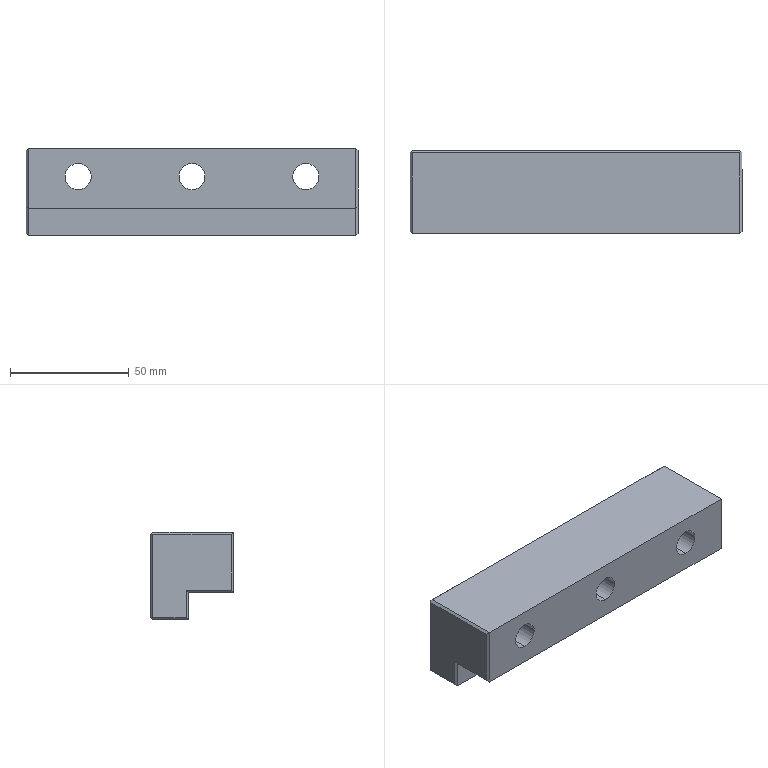Component | SolidWorks | UpperDieShankSeat-1 | 1 solid | 37 faces | box 140 x 35 x 37 mm | volume 135382 mm3 | plane 25 | cylinder 12 | commonest cylinder face diameters 18 x6 11 x6
build123d program:
from build123d import *

# Parameters (mm, degrees)
SKETCH1_W                                        = 140
SKETCH1_H                                        = 140
BOSS_EXTRUDE1_DEPTH                              = 35
SKETCH2_W                                        = 114.165
SKETCH2_H                                        = 44.114
CUT_EXTRUDE1_DEPTH                               = 161.39
SKETCH3_W                                        = 18.069
SKETCH3_H                                        = 21.674
SKETCH3_W_2                                      = 16.574
SKETCH3_H_2                                      = 23.169
CUT_EXTRUDE2_DEPTH                               = 161.39
M10_HEX_SOCKET_HEAD_CAP_SCREW_CBORE1_D           = 11
M10_HEX_SOCKET_HEAD_CAP_SCREW_CBORE1_CBORE_D     = 18
M10_HEX_SOCKET_HEAD_CAP_SCREW_CBORE1_CBORE_DEPTH = 10.6
CHAMFER1_SIZE                                    = 1
CHAMFER2_SIZE                                    = 1
CHAMFER3_SIZE                                    = 1


with BuildPart() as part:
    # Sketch1 → Boss-Extrude1 (new body)
    with BuildSketch(Plane.XY):
        Rectangle(SKETCH1_W, SKETCH1_H)
    extrude(amount=BOSS_EXTRUDE1_DEPTH)

    # Sketch2 → Cut-Extrude1 (cut, through all)
    with BuildSketch(Plane.XZ.offset(70)):
        with Locations((24.082, 18.552)):
            Rectangle(SKETCH2_W, SKETCH2_H)
    extrude(amount=-CUT_EXTRUDE1_DEPTH, mode=Mode.SUBTRACT)

    # Sketch3 → Cut-Extrude2 (cut, through all)
    with BuildSketch(Plane.XZ.offset(70)):
        with Locations((-35.466, 8.163)):
            Rectangle(SKETCH3_W, SKETCH3_H)
        with Locations((35.963, 8.098)):
            Rectangle(SKETCH3_W_2, SKETCH3_H_2)
    extrude(amount=-CUT_EXTRUDE2_DEPTH, mode=Mode.SUBTRACT)

    # M10 Hex Socket Head Cap Screw CBORE1 (through all)
    with Locations(Plane.XY.offset(35)):
        with Locations((-58, 48), (-58, 0), (-58, -48)):
            CounterBoreHole(M10_HEX_SOCKET_HEAD_CAP_SCREW_CBORE1_D / 2, M10_HEX_SOCKET_HEAD_CAP_SCREW_CBORE1_CBORE_D / 2, M10_HEX_SOCKET_HEAD_CAP_SCREW_CBORE1_CBORE_DEPTH)

    # Chamfer1
    chamfer1_edges = [part.edges().sort_by_distance(p)[0] for p in [
        (-33, -70, 27),
        (-38.75, -70, 19),
        (-44.5, -70, 9.5),
        (-57.25, -70, 0),
        (-51.5, -70, 35),
        (-70, -70, 17.5),
    ]]
    chamfer(chamfer1_edges, length=CHAMFER1_SIZE)

    # Chamfer2
    chamfer2_edges = [part.edges().sort_by_distance(p)[0] for p in [
        (-51.5, 70, 35),
        (-33, 70, 27),
        (-57.25, 70, 0),
        (-44.5, 70, 9.5),
        (-38.75, 70, 19),
        (-70, 70, 17.5),
    ]]
    chamfer(chamfer2_edges, length=CHAMFER2_SIZE)

    # Chamfer3
    chamfer3_edges = [part.edges().sort_by_distance(p)[0] for p in [
        (-33, 0, 35),
        (-70, 0, 35),
    ]]
    chamfer(chamfer3_edges, length=CHAMFER3_SIZE)


solid = part.part

# Placed as in the assembly
solid = solid.moved(Location((-177.951, 643.269, 5), (-90, 0, 90)))
STEP:
#1=COLOUR_RGB('',0.7922,0.8196,0.9333);
#2=FILL_AREA_STYLE_COLOUR('',#1);
#3=FILL_AREA_STYLE('',(#2));
#4=SURFACE_STYLE_FILL_AREA(#3);
#5=SURFACE_SIDE_STYLE('',(#4));
#6=SURFACE_STYLE_USAGE(.BOTH.,#5);
#7=PRESENTATION_STYLE_ASSIGNMENT((#6));
#8=CARTESIAN_POINT('',(-8.896,26.286,2.835));
#9=VERTEX_POINT('',#8);
#10=CARTESIAN_POINT('',(-8.896,26.286,2.126));
#11=VERTEX_POINT('',#10);
#12=CARTESIAN_POINT('',(-8.896,26.286,2.48));
#13=DIRECTION('',(-0.,1.,0.));
#14=DIRECTION('',(0.,0.,-1.));
#15=AXIS2_PLACEMENT_3D('',#12,#13,#14);
#16=CIRCLE('',#15,0.3543);
#17=EDGE_CURVE('',#9,#11,#16,.T.);
#18=ORIENTED_EDGE('',*,*,#17,.F.);
#19=CARTESIAN_POINT('',(-8.896,26.704,2.835));
#20=VERTEX_POINT('',#19);
#21=CARTESIAN_POINT('',(-8.896,26.704,2.835));
#22=DIRECTION('',(-0.,1.,0.));
#23=VECTOR('',#22,39.37);
#24=LINE('',#21,#23);
#25=EDGE_CURVE('',#9,#20,#24,.T.);
#26=ORIENTED_EDGE('',*,*,#25,.T.);
#27=CARTESIAN_POINT('',(-8.896,26.704,2.126));
#28=VERTEX_POINT('',#27);
#29=CARTESIAN_POINT('',(-8.896,26.704,2.48));
#30=DIRECTION('',(-0.,1.,0.));
#31=DIRECTION('',(0.,0.,-1.));
#32=AXIS2_PLACEMENT_3D('',#29,#30,#31);
#33=CIRCLE('',#32,0.3543);
#34=EDGE_CURVE('',#20,#28,#33,.T.);
#35=ORIENTED_EDGE('',*,*,#34,.T.);
#36=CARTESIAN_POINT('',(-8.896,26.704,2.126));
#37=DIRECTION('',(-0.,1.,0.));
#38=VECTOR('',#37,39.37);
#39=LINE('',#36,#38);
#40=EDGE_CURVE('',#11,#28,#39,.T.);
#41=ORIENTED_EDGE('',*,*,#40,.F.);
#42=EDGE_LOOP('',(#18,#26,#35,#41));
#43=FACE_OUTER_BOUND('',#42,.T.);
#44=CARTESIAN_POINT('',(-8.896,26.704,2.48));
#45=DIRECTION('',(-0.,1.,0.));
#46=DIRECTION('',(0.,0.,-1.));
#47=AXIS2_PLACEMENT_3D('',#44,#45,#46);
#48=CYLINDRICAL_SURFACE('',#47,0.3543);
#49=ADVANCED_FACE('',(#43),#48,.F.);
#50=CARTESIAN_POINT('',(-8.896,25.326,2.697));
#51=VERTEX_POINT('',#50);
#52=CARTESIAN_POINT('',(-8.896,25.326,2.264));
#53=VERTEX_POINT('',#52);
#54=CARTESIAN_POINT('',(-8.896,25.326,2.48));
#55=DIRECTION('',(-0.,1.,0.));
#56=DIRECTION('',(0.,0.,-1.));
#57=AXIS2_PLACEMENT_3D('',#54,#55,#56);
#58=CIRCLE('',#57,0.2165);
#59=EDGE_CURVE('',#51,#53,#58,.T.);
#60=ORIENTED_EDGE('',*,*,#59,.F.);
#61=CARTESIAN_POINT('',(-8.896,26.286,2.697));
#62=VERTEX_POINT('',#61);
#63=CARTESIAN_POINT('',(-8.896,26.704,2.697));
#64=DIRECTION('',(-0.,1.,0.));
#65=VECTOR('',#64,39.37);
#66=LINE('',#63,#65);
#67=EDGE_CURVE('',#51,#62,#66,.T.);
#68=ORIENTED_EDGE('',*,*,#67,.T.);
#69=CARTESIAN_POINT('',(-8.896,26.286,2.264));
#70=VERTEX_POINT('',#69);
#71=CARTESIAN_POINT('',(-8.896,26.286,2.48));
#72=DIRECTION('',(-0.,1.,0.));
#73=DIRECTION('',(0.,0.,-1.));
#74=AXIS2_PLACEMENT_3D('',#71,#72,#73);
#75=CIRCLE('',#74,0.2165);
#76=EDGE_CURVE('',#62,#70,#75,.T.);
#77=ORIENTED_EDGE('',*,*,#76,.T.);
#78=CARTESIAN_POINT('',(-8.896,26.704,2.264));
#79=DIRECTION('',(-0.,1.,0.));
#80=VECTOR('',#79,39.37);
#81=LINE('',#78,#80);
#82=EDGE_CURVE('',#53,#70,#81,.T.);
#83=ORIENTED_EDGE('',*,*,#82,.F.);
#84=EDGE_LOOP('',(#60,#68,#77,#83));
#85=FACE_OUTER_BOUND('',#84,.T.);
#86=CARTESIAN_POINT('',(-8.896,26.704,2.48));
#87=DIRECTION('',(-0.,1.,0.));
#88=DIRECTION('',(0.,0.,-1.));
#89=AXIS2_PLACEMENT_3D('',#86,#87,#88);
#90=CYLINDRICAL_SURFACE('',#89,0.2165);
#91=ADVANCED_FACE('',(#85),#90,.F.);
#92=CARTESIAN_POINT('',(-7.006,26.286,2.835));
#93=VERTEX_POINT('',#92);
#94=CARTESIAN_POINT('',(-7.006,26.286,2.126));
#95=VERTEX_POINT('',#94);
#96=CARTESIAN_POINT('',(-7.006,26.286,2.48));
#97=DIRECTION('',(-0.,1.,0.));
#98=DIRECTION('',(0.,0.,-1.));
#99=AXIS2_PLACEMENT_3D('',#96,#97,#98);
#100=CIRCLE('',#99,0.3543);
#101=EDGE_CURVE('',#93,#95,#100,.T.);
#102=ORIENTED_EDGE('',*,*,#101,.F.);
#103=CARTESIAN_POINT('',(-7.006,26.704,2.835));
#104=VERTEX_POINT('',#103);
#105=CARTESIAN_POINT('',(-7.006,26.704,2.835));
#106=DIRECTION('',(-0.,1.,0.));
#107=VECTOR('',#106,39.37);
#108=LINE('',#105,#107);
#109=EDGE_CURVE('',#93,#104,#108,.T.);
#110=ORIENTED_EDGE('',*,*,#109,.T.);
#111=CARTESIAN_POINT('',(-7.006,26.704,2.126));
#112=VERTEX_POINT('',#111);
#113=CARTESIAN_POINT('',(-7.006,26.704,2.48));
#114=DIRECTION('',(-0.,1.,0.));
#115=DIRECTION('',(0.,0.,-1.));
#116=AXIS2_PLACEMENT_3D('',#113,#114,#115);
#117=CIRCLE('',#116,0.3543);
#118=EDGE_CURVE('',#104,#112,#117,.T.);
#119=ORIENTED_EDGE('',*,*,#118,.T.);
#120=CARTESIAN_POINT('',(-7.006,26.704,2.126));
#121=DIRECTION('',(-0.,1.,0.));
#122=VECTOR('',#121,39.37);
#123=LINE('',#120,#122);
#124=EDGE_CURVE('',#95,#112,#123,.T.);
#125=ORIENTED_EDGE('',*,*,#124,.F.);
#126=EDGE_LOOP('',(#102,#110,#119,#125));
#127=FACE_OUTER_BOUND('',#126,.T.);
#128=CARTESIAN_POINT('',(-7.006,26.704,2.48));
#129=DIRECTION('',(-0.,1.,0.));
#130=DIRECTION('',(0.,0.,-1.));
#131=AXIS2_PLACEMENT_3D('',#128,#129,#130);
#132=CYLINDRICAL_SURFACE('',#131,0.3543);
#133=ADVANCED_FACE('',(#127),#132,.F.);
#134=CARTESIAN_POINT('',(-7.006,25.326,2.697));
#135=VERTEX_POINT('',#134);
#136=CARTESIAN_POINT('',(-7.006,25.326,2.264));
#137=VERTEX_POINT('',#136);
#138=CARTESIAN_POINT('',(-7.006,25.326,2.48));
#139=DIRECTION('',(-0.,1.,0.));
#140=DIRECTION('',(0.,0.,-1.));
#141=AXIS2_PLACEMENT_3D('',#138,#139,#140);
#142=CIRCLE('',#141,0.2165);
#143=EDGE_CURVE('',#135,#137,#142,.T.);
#144=ORIENTED_EDGE('',*,*,#143,.F.);
#145=CARTESIAN_POINT('',(-7.006,26.286,2.697));
#146=VERTEX_POINT('',#145);
#147=CARTESIAN_POINT('',(-7.006,26.704,2.697));
#148=DIRECTION('',(-0.,1.,0.));
#149=VECTOR('',#148,39.37);
#150=LINE('',#147,#149);
#151=EDGE_CURVE('',#135,#146,#150,.T.);
#152=ORIENTED_EDGE('',*,*,#151,.T.);
#153=CARTESIAN_POINT('',(-7.006,26.286,2.264));
#154=VERTEX_POINT('',#153);
#155=CARTESIAN_POINT('',(-7.006,26.286,2.48));
#156=DIRECTION('',(-0.,1.,0.));
#157=DIRECTION('',(0.,0.,-1.));
#158=AXIS2_PLACEMENT_3D('',#155,#156,#157);
#159=CIRCLE('',#158,0.2165);
#160=EDGE_CURVE('',#146,#154,#159,.T.);
#161=ORIENTED_EDGE('',*,*,#160,.T.);
#162=CARTESIAN_POINT('',(-7.006,26.704,2.264));
#163=DIRECTION('',(-0.,1.,0.));
#164=VECTOR('',#163,39.37);
#165=LINE('',#162,#164);
#166=EDGE_CURVE('',#137,#154,#165,.T.);
#167=ORIENTED_EDGE('',*,*,#166,.F.);
#168=EDGE_LOOP('',(#144,#152,#161,#167));
#169=FACE_OUTER_BOUND('',#168,.T.);
#170=CARTESIAN_POINT('',(-7.006,26.704,2.48));
#171=DIRECTION('',(-0.,1.,0.));
#172=DIRECTION('',(0.,0.,-1.));
#173=AXIS2_PLACEMENT_3D('',#170,#171,#172);
#174=CYLINDRICAL_SURFACE('',#173,0.2165);
#175=ADVANCED_FACE('',(#169),#174,.F.);
#176=CARTESIAN_POINT('',(-5.116,26.286,2.835));
#177=VERTEX_POINT('',#176);
#178=CARTESIAN_POINT('',(-5.116,26.286,2.126));
#179=VERTEX_POINT('',#178);
#180=CARTESIAN_POINT('',(-5.116,26.286,2.48));
#181=DIRECTION('',(-0.,1.,0.));
#182=DIRECTION('',(0.,0.,-1.));
#183=AXIS2_PLACEMENT_3D('',#180,#181,#182);
#184=CIRCLE('',#183,0.3543);
#185=EDGE_CURVE('',#177,#179,#184,.T.);
#186=ORIENTED_EDGE('',*,*,#185,.F.);
#187=CARTESIAN_POINT('',(-5.116,26.704,2.835));
#188=VERTEX_POINT('',#187);
#189=CARTESIAN_POINT('',(-5.116,26.704,2.835));
#190=DIRECTION('',(-0.,1.,0.));
#191=VECTOR('',#190,39.37);
#192=LINE('',#189,#191);
#193=EDGE_CURVE('',#177,#188,#192,.T.);
#194=ORIENTED_EDGE('',*,*,#193,.T.);
#195=CARTESIAN_POINT('',(-5.116,26.704,2.126));
#196=VERTEX_POINT('',#195);
#197=CARTESIAN_POINT('',(-5.116,26.704,2.48));
#198=DIRECTION('',(-0.,1.,0.));
#199=DIRECTION('',(0.,0.,-1.));
#200=AXIS2_PLACEMENT_3D('',#197,#198,#199);
#201=CIRCLE('',#200,0.3543);
#202=EDGE_CURVE('',#188,#196,#201,.T.);
#203=ORIENTED_EDGE('',*,*,#202,.T.);
#204=CARTESIAN_POINT('',(-5.116,26.704,2.126));
#205=DIRECTION('',(-0.,1.,0.));
#206=VECTOR('',#205,39.37);
#207=LINE('',#204,#206);
#208=EDGE_CURVE('',#179,#196,#207,.T.);
#209=ORIENTED_EDGE('',*,*,#208,.F.);
#210=EDGE_LOOP('',(#186,#194,#203,#209));
#211=FACE_OUTER_BOUND('',#210,.T.);
#212=CARTESIAN_POINT('',(-5.116,26.704,2.48));
#213=DIRECTION('',(-0.,1.,0.));
#214=DIRECTION('',(0.,0.,-1.));
#215=AXIS2_PLACEMENT_3D('',#212,#213,#214);
#216=CYLINDRICAL_SURFACE('',#215,0.3543);
#217=ADVANCED_FACE('',(#211),#216,.F.);
#218=CARTESIAN_POINT('',(-5.116,25.326,2.697));
#219=VERTEX_POINT('',#218);
#220=CARTESIAN_POINT('',(-5.116,25.326,2.264));
#221=VERTEX_POINT('',#220);
#222=CARTESIAN_POINT('',(-5.116,25.326,2.48));
#223=DIRECTION('',(-0.,1.,0.));
#224=DIRECTION('',(0.,0.,-1.));
#225=AXIS2_PLACEMENT_3D('',#222,#223,#224);
#226=CIRCLE('',#225,0.2165);
#227=EDGE_CURVE('',#219,#221,#226,.T.);
#228=ORIENTED_EDGE('',*,*,#227,.F.);
#229=CARTESIAN_POINT('',(-5.116,26.286,2.697));
#230=VERTEX_POINT('',#229);
#231=CARTESIAN_POINT('',(-5.116,26.704,2.697));
#232=DIRECTION('',(-0.,1.,0.));
#233=VECTOR('',#232,39.37);
#234=LINE('',#231,#233);
#235=EDGE_CURVE('',#219,#230,#234,.T.);
#236=ORIENTED_EDGE('',*,*,#235,.T.);
#237=CARTESIAN_POINT('',(-5.116,26.286,2.264));
#238=VERTEX_POINT('',#237);
#239=CARTESIAN_POINT('',(-5.116,26.286,2.48));
#240=DIRECTION('',(-0.,1.,0.));
#241=DIRECTION('',(0.,0.,-1.));
#242=AXIS2_PLACEMENT_3D('',#239,#240,#241);
#243=CIRCLE('',#242,0.2165);
#244=EDGE_CURVE('',#230,#238,#243,.T.);
#245=ORIENTED_EDGE('',*,*,#244,.T.);
#246=CARTESIAN_POINT('',(-5.116,26.704,2.264));
#247=DIRECTION('',(-0.,1.,0.));
#248=VECTOR('',#247,39.37);
#249=LINE('',#246,#248);
#250=EDGE_CURVE('',#221,#238,#249,.T.);
#251=ORIENTED_EDGE('',*,*,#250,.F.);
#252=EDGE_LOOP('',(#228,#236,#245,#251));
#253=FACE_OUTER_BOUND('',#252,.T.);
#254=CARTESIAN_POINT('',(-5.116,26.704,2.48));
#255=DIRECTION('',(-0.,1.,0.));
#256=DIRECTION('',(0.,0.,-1.));
#257=AXIS2_PLACEMENT_3D('',#254,#255,#256);
#258=CYLINDRICAL_SURFACE('',#257,0.2165);
#259=ADVANCED_FACE('',(#253),#258,.F.);
#260=CARTESIAN_POINT('',(-4.289,25.326,2.953));
#261=VERTEX_POINT('',#260);
#262=CARTESIAN_POINT('',(-4.289,26.664,2.953));
#263=VERTEX_POINT('',#262);
#264=CARTESIAN_POINT('',(-4.289,26.704,2.953));
#265=DIRECTION('',(-0.,1.,0.));
#266=VECTOR('',#265,39.37);
#267=LINE('',#264,#266);
#268=EDGE_CURVE('',#261,#263,#267,.T.);
#269=ORIENTED_EDGE('',*,*,#268,.T.);
#270=CARTESIAN_POINT('',(-9.722,26.664,2.953));
#271=VERTEX_POINT('',#270);
#272=CARTESIAN_POINT('',(-9.722,26.664,2.953));
#273=DIRECTION('',(-1.,-0.,-0.));
#274=VECTOR('',#273,39.37);
#275=LINE('',#272,#274);
#276=EDGE_CURVE('',#263,#271,#275,.T.);
#277=ORIENTED_EDGE('',*,*,#276,.T.);
#278=CARTESIAN_POINT('',(-9.722,25.326,2.953));
#279=VERTEX_POINT('',#278);
#280=CARTESIAN_POINT('',(-9.722,26.704,2.953));
#281=DIRECTION('',(0.,-1.,-0.));
#282=VECTOR('',#281,39.37);
#283=LINE('',#280,#282);
#284=EDGE_CURVE('',#271,#279,#283,.T.);
#285=ORIENTED_EDGE('',*,*,#284,.T.);
#286=CARTESIAN_POINT('',(-9.762,25.326,2.953));
#287=DIRECTION('',(1.,0.,0.));
#288=VECTOR('',#287,39.37);
#289=LINE('',#286,#288);
#290=EDGE_CURVE('',#279,#261,#289,.T.);
#291=ORIENTED_EDGE('',*,*,#290,.T.);
#292=EDGE_LOOP('',(#269,#277,#285,#291));
#293=FACE_OUTER_BOUND('',#292,.T.);
#294=CARTESIAN_POINT('',(-9.762,26.704,2.953));
#295=DIRECTION('',(0.,0.,-1.));
#296=DIRECTION('',(0.,-1.,-0.));
#297=AXIS2_PLACEMENT_3D('',#294,#295,#296);
#298=PLANE('',#297);
#299=ADVANCED_FACE('',(#293),#298,.F.);
#300=CARTESIAN_POINT('',(-4.25,26.664,1.535));
#301=VERTEX_POINT('',#300);
#302=CARTESIAN_POINT('',(-4.25,26.664,2.913));
#303=VERTEX_POINT('',#302);
#304=CARTESIAN_POINT('',(-4.25,26.664,2.953));
#305=DIRECTION('',(-0.,-0.,1.));
#306=VECTOR('',#305,39.37);
#307=LINE('',#304,#306);
#308=EDGE_CURVE('',#301,#303,#307,.T.);
#309=ORIENTED_EDGE('',*,*,#308,.T.);
#310=CARTESIAN_POINT('',(-4.25,25.365,2.913));
#311=VERTEX_POINT('',#310);
#312=CARTESIAN_POINT('',(-4.25,26.704,2.913));
#313=DIRECTION('',(0.,-1.,-0.));
#314=VECTOR('',#313,39.37);
#315=LINE('',#312,#314);
#316=EDGE_CURVE('',#303,#311,#315,.T.);
#317=ORIENTED_EDGE('',*,*,#316,.T.);
#318=CARTESIAN_POINT('',(-4.25,25.365,1.988));
#319=VERTEX_POINT('',#318);
#320=CARTESIAN_POINT('',(-4.25,25.365,2.953));
#321=DIRECTION('',(0.,0.,-1.));
#322=VECTOR('',#321,39.37);
#323=LINE('',#320,#322);
#324=EDGE_CURVE('',#311,#319,#323,.T.);
#325=ORIENTED_EDGE('',*,*,#324,.T.);
#326=CARTESIAN_POINT('',(-4.25,26.113,1.988));
#327=VERTEX_POINT('',#326);
#328=CARTESIAN_POINT('',(-4.25,26.704,1.988));
#329=DIRECTION('',(-0.,1.,0.));
#330=VECTOR('',#329,39.37);
#331=LINE('',#328,#330);
#332=EDGE_CURVE('',#319,#327,#331,.T.);
#333=ORIENTED_EDGE('',*,*,#332,.T.);
#334=CARTESIAN_POINT('',(-4.25,26.113,1.535));
#335=VERTEX_POINT('',#334);
#336=CARTESIAN_POINT('',(-4.25,26.113,2.953));
#337=DIRECTION('',(0.,0.,-1.));
#338=VECTOR('',#337,39.37);
#339=LINE('',#336,#338);
#340=EDGE_CURVE('',#327,#335,#339,.T.);
#341=ORIENTED_EDGE('',*,*,#340,.T.);
#342=CARTESIAN_POINT('',(-4.25,26.704,1.535));
#343=DIRECTION('',(-0.,1.,0.));
#344=VECTOR('',#343,39.37);
#345=LINE('',#342,#344);
#346=EDGE_CURVE('',#335,#301,#345,.T.);
#347=ORIENTED_EDGE('',*,*,#346,.T.);
#348=EDGE_LOOP('',(#309,#317,#325,#333,#341,#347));
#349=FACE_OUTER_BOUND('',#348,.T.);
#350=CARTESIAN_POINT('',(-4.25,26.704,2.953));
#351=DIRECTION('',(-1.,-0.,-0.));
#352=DIRECTION('',(-0.,1.,0.));
#353=AXIS2_PLACEMENT_3D('',#350,#351,#352);
#354=PLANE('',#353);
#355=ADVANCED_FACE('',(#349),#354,.F.);
#356=CARTESIAN_POINT('',(-9.762,26.664,2.913));
#357=VERTEX_POINT('',#356);
#358=CARTESIAN_POINT('',(-9.762,26.664,1.535));
#359=VERTEX_POINT('',#358);
#360=CARTESIAN_POINT('',(-9.762,26.664,1.496));
#361=DIRECTION('',(0.,0.,-1.));
#362=VECTOR('',#361,39.37);
#363=LINE('',#360,#362);
#364=EDGE_CURVE('',#357,#359,#363,.T.);
#365=ORIENTED_EDGE('',*,*,#364,.T.);
#366=CARTESIAN_POINT('',(-9.762,26.113,1.535));
#367=VERTEX_POINT('',#366);
#368=CARTESIAN_POINT('',(-9.762,26.704,1.535));
#369=DIRECTION('',(0.,-1.,-0.));
#370=VECTOR('',#369,39.37);
#371=LINE('',#368,#370);
#372=EDGE_CURVE('',#359,#367,#371,.T.);
#373=ORIENTED_EDGE('',*,*,#372,.T.);
#374=CARTESIAN_POINT('',(-9.762,26.113,1.988));
#375=VERTEX_POINT('',#374);
#376=CARTESIAN_POINT('',(-9.762,26.113,2.953));
#377=DIRECTION('',(-0.,-0.,1.));
#378=VECTOR('',#377,39.37);
#379=LINE('',#376,#378);
#380=EDGE_CURVE('',#367,#375,#379,.T.);
#381=ORIENTED_EDGE('',*,*,#380,.T.);
#382=CARTESIAN_POINT('',(-9.762,25.365,1.988));
#383=VERTEX_POINT('',#382);
#384=CARTESIAN_POINT('',(-9.762,26.704,1.988));
#385=DIRECTION('',(0.,-1.,-0.));
#386=VECTOR('',#385,39.37);
#387=LINE('',#384,#386);
#388=EDGE_CURVE('',#375,#383,#387,.T.);
#389=ORIENTED_EDGE('',*,*,#388,.T.);
#390=CARTESIAN_POINT('',(-9.762,25.365,2.913));
#391=VERTEX_POINT('',#390);
#392=CARTESIAN_POINT('',(-9.762,25.365,2.953));
#393=DIRECTION('',(-0.,-0.,1.));
#394=VECTOR('',#393,39.37);
#395=LINE('',#392,#394);
#396=EDGE_CURVE('',#383,#391,#395,.T.);
#397=ORIENTED_EDGE('',*,*,#396,.T.);
#398=CARTESIAN_POINT('',(-9.762,26.704,2.913));
#399=DIRECTION('',(-0.,1.,0.));
#400=VECTOR('',#399,39.37);
#401=LINE('',#398,#400);
#402=EDGE_CURVE('',#391,#357,#401,.T.);
#403=ORIENTED_EDGE('',*,*,#402,.T.);
#404=EDGE_LOOP('',(#365,#373,#381,#389,#397,#403));
#405=FACE_OUTER_BOUND('',#404,.T.);
#406=CARTESIAN_POINT('',(-9.762,26.704,2.953));
#407=DIRECTION('',(1.,0.,0.));
#408=DIRECTION('',(0.,-1.,-0.));
#409=AXIS2_PLACEMENT_3D('',#406,#407,#408);
#410=PLANE('',#409);
#411=ADVANCED_FACE('',(#405),#410,.F.);
#412=CARTESIAN_POINT('',(-8.896,26.704,2.48));
#413=DIRECTION('',(-0.,1.,0.));
#414=DIRECTION('',(0.,0.,-1.));
#415=AXIS2_PLACEMENT_3D('',#412,#413,#414);
#416=CIRCLE('',#415,0.3543);
#417=EDGE_CURVE('',#28,#20,#416,.T.);
#418=ORIENTED_EDGE('',*,*,#417,.F.);
#419=ORIENTED_EDGE('',*,*,#34,.F.);
#420=EDGE_LOOP('',(#418,#419));
#421=FACE_BOUND('',#420,.T.);
#422=CARTESIAN_POINT('',(-7.006,26.704,2.48));
#423=DIRECTION('',(-0.,1.,0.));
#424=DIRECTION('',(0.,0.,-1.));
#425=AXIS2_PLACEMENT_3D('',#422,#423,#424);
#426=CIRCLE('',#425,0.3543);
#427=EDGE_CURVE('',#112,#104,#426,.T.);
#428=ORIENTED_EDGE('',*,*,#427,.F.);
#429=ORIENTED_EDGE('',*,*,#118,.F.);
#430=EDGE_LOOP('',(#428,#429));
#431=FACE_BOUND('',#430,.T.);
#432=CARTESIAN_POINT('',(-5.116,26.704,2.48));
#433=DIRECTION('',(-0.,1.,0.));
#434=DIRECTION('',(0.,0.,-1.));
#435=AXIS2_PLACEMENT_3D('',#432,#433,#434);
#436=CIRCLE('',#435,0.3543);
#437=EDGE_CURVE('',#196,#188,#436,.T.);
#438=ORIENTED_EDGE('',*,*,#437,.F.);
#439=ORIENTED_EDGE('',*,*,#202,.F.);
#440=EDGE_LOOP('',(#438,#439));
#441=FACE_BOUND('',#440,.T.);
#442=CARTESIAN_POINT('',(-9.722,26.704,1.535));
#443=VERTEX_POINT('',#442);
#444=CARTESIAN_POINT('',(-9.722,26.704,2.913));
#445=VERTEX_POINT('',#444);
#446=CARTESIAN_POINT('',(-9.722,26.704,2.953));
#447=DIRECTION('',(-0.,-0.,1.));
#448=VECTOR('',#447,39.37);
#449=LINE('',#446,#448);
#450=EDGE_CURVE('',#443,#445,#449,.T.);
#451=ORIENTED_EDGE('',*,*,#450,.T.);
#452=CARTESIAN_POINT('',(-4.289,26.704,2.913));
#453=VERTEX_POINT('',#452);
#454=CARTESIAN_POINT('',(-4.289,26.704,2.913));
#455=DIRECTION('',(1.,0.,0.));
#456=VECTOR('',#455,39.37);
#457=LINE('',#454,#456);
#458=EDGE_CURVE('',#445,#453,#457,.T.);
#459=ORIENTED_EDGE('',*,*,#458,.T.);
#460=CARTESIAN_POINT('',(-4.289,26.704,1.535));
#461=VERTEX_POINT('',#460);
#462=CARTESIAN_POINT('',(-4.289,26.704,1.496));
#463=DIRECTION('',(0.,0.,-1.));
#464=VECTOR('',#463,39.37);
#465=LINE('',#462,#464);
#466=EDGE_CURVE('',#453,#461,#465,.T.);
#467=ORIENTED_EDGE('',*,*,#466,.T.);
#468=CARTESIAN_POINT('',(-9.722,26.704,1.535));
#469=DIRECTION('',(-1.,-0.,-0.));
#470=VECTOR('',#469,39.37);
#471=LINE('',#468,#470);
#472=EDGE_CURVE('',#461,#443,#471,.T.);
#473=ORIENTED_EDGE('',*,*,#472,.T.);
#474=EDGE_LOOP('',(#451,#459,#467,#473));
#475=FACE_OUTER_BOUND('',#474,.T.);
#476=CARTESIAN_POINT('',(-7.006,26.704,0.1969));
#477=DIRECTION('',(-0.,1.,0.));
#478=DIRECTION('',(0.,0.,-1.));
#479=AXIS2_PLACEMENT_3D('',#476,#477,#478);
#480=PLANE('',#479);
#481=ADVANCED_FACE('',(#421,#431,#441,#475),#480,.T.);
#482=CARTESIAN_POINT('',(-8.896,25.326,2.48));
#483=DIRECTION('',(-0.,1.,0.));
#484=DIRECTION('',(0.,0.,-1.));
#485=AXIS2_PLACEMENT_3D('',#482,#483,#484);
#486=CIRCLE('',#485,0.2165);
#487=EDGE_CURVE('',#53,#51,#486,.T.);
#488=ORIENTED_EDGE('',*,*,#487,.T.);
#489=ORIENTED_EDGE('',*,*,#59,.T.);
#490=EDGE_LOOP('',(#488,#489));
#491=FACE_BOUND('',#490,.T.);
#492=CARTESIAN_POINT('',(-7.006,25.326,2.48));
#493=DIRECTION('',(-0.,1.,0.));
#494=DIRECTION('',(0.,0.,-1.));
#495=AXIS2_PLACEMENT_3D('',#492,#493,#494);
#496=CIRCLE('',#495,0.2165);
#497=EDGE_CURVE('',#137,#135,#496,.T.);
#498=ORIENTED_EDGE('',*,*,#497,.T.);
#499=ORIENTED_EDGE('',*,*,#143,.T.);
#500=EDGE_LOOP('',(#498,#499));
#501=FACE_BOUND('',#500,.T.);
#502=CARTESIAN_POINT('',(-5.116,25.326,2.48));
#503=DIRECTION('',(-0.,1.,0.));
#504=DIRECTION('',(0.,0.,-1.));
#505=AXIS2_PLACEMENT_3D('',#502,#503,#504);
#506=CIRCLE('',#505,0.2165);
#507=EDGE_CURVE('',#221,#219,#506,.T.);
#508=ORIENTED_EDGE('',*,*,#507,.T.);
#509=ORIENTED_EDGE('',*,*,#227,.T.);
#510=EDGE_LOOP('',(#508,#509));
#511=FACE_BOUND('',#510,.T.);
#512=ORIENTED_EDGE('',*,*,#290,.F.);
#513=CARTESIAN_POINT('',(-9.722,25.326,1.949));
#514=VERTEX_POINT('',#513);
#515=CARTESIAN_POINT('',(-9.722,25.326,0.1969));
#516=DIRECTION('',(0.,0.,-1.));
#517=VECTOR('',#516,39.37);
#518=LINE('',#515,#517);
#519=EDGE_CURVE('',#279,#514,#518,.T.);
#520=ORIENTED_EDGE('',*,*,#519,.T.);
#521=CARTESIAN_POINT('',(-4.289,25.326,1.949));
#522=VERTEX_POINT('',#521);
#523=CARTESIAN_POINT('',(-7.006,25.326,1.949));
#524=DIRECTION('',(1.,0.,0.));
#525=VECTOR('',#524,39.37);
#526=LINE('',#523,#525);
#527=EDGE_CURVE('',#514,#522,#526,.T.);
#528=ORIENTED_EDGE('',*,*,#527,.T.);
#529=CARTESIAN_POINT('',(-4.289,25.326,0.1969));
#530=DIRECTION('',(-0.,-0.,1.));
#531=VECTOR('',#530,39.37);
#532=LINE('',#529,#531);
#533=EDGE_CURVE('',#522,#261,#532,.T.);
#534=ORIENTED_EDGE('',*,*,#533,.T.);
#535=EDGE_LOOP('',(#512,#520,#528,#534));
#536=FACE_OUTER_BOUND('',#535,.T.);
#537=CARTESIAN_POINT('',(-7.006,25.326,0.1969));
#538=DIRECTION('',(-0.,1.,0.));
#539=DIRECTION('',(0.,0.,-1.));
#540=AXIS2_PLACEMENT_3D('',#537,#538,#539);
#541=PLANE('',#540);
#542=ADVANCED_FACE('',(#491,#501,#511,#536),#541,.F.);
#543=CARTESIAN_POINT('',(-9.722,26.074,1.496));
#544=VERTEX_POINT('',#543);
#545=CARTESIAN_POINT('',(-9.722,26.664,1.496));
#546=VERTEX_POINT('',#545);
#547=CARTESIAN_POINT('',(-9.722,26.924,1.496));
#548=DIRECTION('',(-0.,1.,0.));
#549=VECTOR('',#548,39.37);
#550=LINE('',#547,#549);
#551=EDGE_CURVE('',#544,#546,#550,.T.);
#552=ORIENTED_EDGE('',*,*,#551,.T.);
#553=CARTESIAN_POINT('',(-4.289,26.664,1.496));
#554=VERTEX_POINT('',#553);
#555=CARTESIAN_POINT('',(-4.289,26.664,1.496));
#556=DIRECTION('',(1.,0.,0.));
#557=VECTOR('',#556,39.37);
#558=LINE('',#555,#557);
#559=EDGE_CURVE('',#546,#554,#558,.T.);
#560=ORIENTED_EDGE('',*,*,#559,.T.);
#561=CARTESIAN_POINT('',(-4.289,26.074,1.496));
#562=VERTEX_POINT('',#561);
#563=CARTESIAN_POINT('',(-4.289,26.924,1.496));
#564=DIRECTION('',(0.,-1.,-0.));
#565=VECTOR('',#564,39.37);
#566=LINE('',#563,#565);
#567=EDGE_CURVE('',#554,#562,#566,.T.);
#568=ORIENTED_EDGE('',*,*,#567,.T.);
#569=CARTESIAN_POINT('',(-9.762,26.074,1.496));
#570=DIRECTION('',(-1.,-0.,-0.));
#571=VECTOR('',#570,39.37);
#572=LINE('',#569,#571);
#573=EDGE_CURVE('',#562,#544,#572,.T.);
#574=ORIENTED_EDGE('',*,*,#573,.T.);
#575=EDGE_LOOP('',(#552,#560,#568,#574));
#576=FACE_OUTER_BOUND('',#575,.T.);
#577=CARTESIAN_POINT('',(-9.762,26.924,1.496));
#578=DIRECTION('',(-0.,-0.,1.));
#579=DIRECTION('',(-0.,1.,0.));
#580=AXIS2_PLACEMENT_3D('',#577,#578,#579);
#581=PLANE('',#580);
#582=ADVANCED_FACE('',(#576),#581,.F.);
#583=ORIENTED_EDGE('',*,*,#527,.F.);
#584=CARTESIAN_POINT('',(-9.722,26.074,1.949));
#585=VERTEX_POINT('',#584);
#586=CARTESIAN_POINT('',(-9.722,26.074,1.949));
#587=DIRECTION('',(-0.,1.,0.));
#588=VECTOR('',#587,39.37);
#589=LINE('',#586,#588);
#590=EDGE_CURVE('',#514,#585,#589,.T.);
#591=ORIENTED_EDGE('',*,*,#590,.T.);
#592=CARTESIAN_POINT('',(-4.289,26.074,1.949));
#593=VERTEX_POINT('',#592);
#594=CARTESIAN_POINT('',(-9.762,26.074,1.949));
#595=DIRECTION('',(1.,0.,0.));
#596=VECTOR('',#595,39.37);
#597=LINE('',#594,#596);
#598=EDGE_CURVE('',#585,#593,#597,.T.);
#599=ORIENTED_EDGE('',*,*,#598,.T.);
#600=CARTESIAN_POINT('',(-4.289,26.074,1.949));
#601=DIRECTION('',(0.,-1.,-0.));
#602=VECTOR('',#601,39.37);
#603=LINE('',#600,#602);
#604=EDGE_CURVE('',#593,#522,#603,.T.);
#605=ORIENTED_EDGE('',*,*,#604,.T.);
#606=EDGE_LOOP('',(#583,#591,#599,#605));
#607=FACE_OUTER_BOUND('',#606,.T.);
#608=CARTESIAN_POINT('',(-9.762,26.074,1.949));
#609=DIRECTION('',(-0.,-0.,1.));
#610=DIRECTION('',(-0.,1.,0.));
#611=AXIS2_PLACEMENT_3D('',#608,#609,#610);
#612=PLANE('',#611);
#613=ADVANCED_FACE('',(#607),#612,.F.);
#614=ORIENTED_EDGE('',*,*,#598,.F.);
#615=CARTESIAN_POINT('',(-9.722,26.074,1.237));
#616=DIRECTION('',(0.,0.,-1.));
#617=VECTOR('',#616,39.37);
#618=LINE('',#615,#617);
#619=EDGE_CURVE('',#585,#544,#618,.T.);
#620=ORIENTED_EDGE('',*,*,#619,.T.);
#621=ORIENTED_EDGE('',*,*,#573,.F.);
#622=CARTESIAN_POINT('',(-4.289,26.074,1.237));
#623=DIRECTION('',(-0.,-0.,1.));
#624=VECTOR('',#623,39.37);
#625=LINE('',#622,#624);
#626=EDGE_CURVE('',#562,#593,#625,.T.);
#627=ORIENTED_EDGE('',*,*,#626,.T.);
#628=EDGE_LOOP('',(#614,#620,#621,#627));
#629=FACE_OUTER_BOUND('',#628,.T.);
#630=CARTESIAN_POINT('',(-9.762,26.074,1.237));
#631=DIRECTION('',(-0.,1.,0.));
#632=DIRECTION('',(0.,0.,-1.));
#633=AXIS2_PLACEMENT_3D('',#630,#631,#632);
#634=PLANE('',#633);
#635=ADVANCED_FACE('',(#629),#634,.F.);
#636=ORIENTED_EDGE('',*,*,#235,.F.);
#637=ORIENTED_EDGE('',*,*,#507,.F.);
#638=ORIENTED_EDGE('',*,*,#250,.T.);
#639=CARTESIAN_POINT('',(-5.116,26.286,2.48));
#640=DIRECTION('',(-0.,1.,0.));
#641=DIRECTION('',(0.,0.,-1.));
#642=AXIS2_PLACEMENT_3D('',#639,#640,#641);
#643=CIRCLE('',#642,0.2165);
#644=EDGE_CURVE('',#238,#230,#643,.T.);
#645=ORIENTED_EDGE('',*,*,#644,.T.);
#646=EDGE_LOOP('',(#636,#637,#638,#645));
#647=FACE_OUTER_BOUND('',#646,.T.);
#648=CARTESIAN_POINT('',(-5.116,26.704,2.48));
#649=DIRECTION('',(-0.,1.,0.));
#650=DIRECTION('',(0.,0.,-1.));
#651=AXIS2_PLACEMENT_3D('',#648,#649,#650);
#652=CYLINDRICAL_SURFACE('',#651,0.2165);
#653=ADVANCED_FACE('',(#647),#652,.F.);
#654=ORIENTED_EDGE('',*,*,#644,.F.);
#655=ORIENTED_EDGE('',*,*,#244,.F.);
#656=EDGE_LOOP('',(#654,#655));
#657=FACE_BOUND('',#656,.T.);
#658=CARTESIAN_POINT('',(-5.116,26.286,2.48));
#659=DIRECTION('',(-0.,1.,0.));
#660=DIRECTION('',(0.,0.,-1.));
#661=AXIS2_PLACEMENT_3D('',#658,#659,#660);
#662=CIRCLE('',#661,0.3543);
#663=EDGE_CURVE('',#179,#177,#662,.T.);
#664=ORIENTED_EDGE('',*,*,#663,.T.);
#665=ORIENTED_EDGE('',*,*,#185,.T.);
#666=EDGE_LOOP('',(#664,#665));
#667=FACE_OUTER_BOUND('',#666,.T.);
#668=CARTESIAN_POINT('',(-5.116,26.286,2.264));
#669=DIRECTION('',(0.,-1.,-0.));
#670=DIRECTION('',(-0.,-0.,1.));
#671=AXIS2_PLACEMENT_3D('',#668,#669,#670);
#672=PLANE('',#671);
#673=ADVANCED_FACE('',(#657,#667),#672,.F.);
#674=ORIENTED_EDGE('',*,*,#193,.F.);
#675=ORIENTED_EDGE('',*,*,#663,.F.);
#676=ORIENTED_EDGE('',*,*,#208,.T.);
#677=ORIENTED_EDGE('',*,*,#437,.T.);
#678=EDGE_LOOP('',(#674,#675,#676,#677));
#679=FACE_OUTER_BOUND('',#678,.T.);
#680=CARTESIAN_POINT('',(-5.116,26.704,2.48));
#681=DIRECTION('',(-0.,1.,0.));
#682=DIRECTION('',(0.,0.,-1.));
#683=AXIS2_PLACEMENT_3D('',#680,#681,#682);
#684=CYLINDRICAL_SURFACE('',#683,0.3543);
#685=ADVANCED_FACE('',(#679),#684,.F.);
#686=ORIENTED_EDGE('',*,*,#151,.F.);
#687=ORIENTED_EDGE('',*,*,#497,.F.);
#688=ORIENTED_EDGE('',*,*,#166,.T.);
#689=CARTESIAN_POINT('',(-7.006,26.286,2.48));
#690=DIRECTION('',(-0.,1.,0.));
#691=DIRECTION('',(0.,0.,-1.));
#692=AXIS2_PLACEMENT_3D('',#689,#690,#691);
#693=CIRCLE('',#692,0.2165);
#694=EDGE_CURVE('',#154,#146,#693,.T.);
#695=ORIENTED_EDGE('',*,*,#694,.T.);
#696=EDGE_LOOP('',(#686,#687,#688,#695));
#697=FACE_OUTER_BOUND('',#696,.T.);
#698=CARTESIAN_POINT('',(-7.006,26.704,2.48));
#699=DIRECTION('',(-0.,1.,0.));
#700=DIRECTION('',(0.,0.,-1.));
#701=AXIS2_PLACEMENT_3D('',#698,#699,#700);
#702=CYLINDRICAL_SURFACE('',#701,0.2165);
#703=ADVANCED_FACE('',(#697),#702,.F.);
#704=ORIENTED_EDGE('',*,*,#694,.F.);
#705=ORIENTED_EDGE('',*,*,#160,.F.);
#706=EDGE_LOOP('',(#704,#705));
#707=FACE_BOUND('',#706,.T.);
#708=CARTESIAN_POINT('',(-7.006,26.286,2.48));
#709=DIRECTION('',(-0.,1.,0.));
#710=DIRECTION('',(0.,0.,-1.));
#711=AXIS2_PLACEMENT_3D('',#708,#709,#710);
#712=CIRCLE('',#711,0.3543);
#713=EDGE_CURVE('',#95,#93,#712,.T.);
#714=ORIENTED_EDGE('',*,*,#713,.T.);
#715=ORIENTED_EDGE('',*,*,#101,.T.);
#716=EDGE_LOOP('',(#714,#715));
#717=FACE_OUTER_BOUND('',#716,.T.);
#718=CARTESIAN_POINT('',(-7.006,26.286,2.264));
#719=DIRECTION('',(0.,-1.,-0.));
#720=DIRECTION('',(-0.,-0.,1.));
#721=AXIS2_PLACEMENT_3D('',#718,#719,#720);
#722=PLANE('',#721);
#723=ADVANCED_FACE('',(#707,#717),#722,.F.);
#724=ORIENTED_EDGE('',*,*,#109,.F.);
#725=ORIENTED_EDGE('',*,*,#713,.F.);
#726=ORIENTED_EDGE('',*,*,#124,.T.);
#727=ORIENTED_EDGE('',*,*,#427,.T.);
#728=EDGE_LOOP('',(#724,#725,#726,#727));
#729=FACE_OUTER_BOUND('',#728,.T.);
#730=CARTESIAN_POINT('',(-7.006,26.704,2.48));
#731=DIRECTION('',(-0.,1.,0.));
#732=DIRECTION('',(0.,0.,-1.));
#733=AXIS2_PLACEMENT_3D('',#730,#731,#732);
#734=CYLINDRICAL_SURFACE('',#733,0.3543);
#735=ADVANCED_FACE('',(#729),#734,.F.);
#736=ORIENTED_EDGE('',*,*,#67,.F.);
#737=ORIENTED_EDGE('',*,*,#487,.F.);
#738=ORIENTED_EDGE('',*,*,#82,.T.);
#739=CARTESIAN_POINT('',(-8.896,26.286,2.48));
#740=DIRECTION('',(-0.,1.,0.));
#741=DIRECTION('',(0.,0.,-1.));
#742=AXIS2_PLACEMENT_3D('',#739,#740,#741);
#743=CIRCLE('',#742,0.2165);
#744=EDGE_CURVE('',#70,#62,#743,.T.);
#745=ORIENTED_EDGE('',*,*,#744,.T.);
#746=EDGE_LOOP('',(#736,#737,#738,#745));
#747=FACE_OUTER_BOUND('',#746,.T.);
#748=CARTESIAN_POINT('',(-8.896,26.704,2.48));
#749=DIRECTION('',(-0.,1.,0.));
#750=DIRECTION('',(0.,0.,-1.));
#751=AXIS2_PLACEMENT_3D('',#748,#749,#750);
#752=CYLINDRICAL_SURFACE('',#751,0.2165);
#753=ADVANCED_FACE('',(#747),#752,.F.);
#754=ORIENTED_EDGE('',*,*,#744,.F.);
#755=ORIENTED_EDGE('',*,*,#76,.F.);
#756=EDGE_LOOP('',(#754,#755));
#757=FACE_BOUND('',#756,.T.);
#758=CARTESIAN_POINT('',(-8.896,26.286,2.48));
#759=DIRECTION('',(-0.,1.,0.));
#760=DIRECTION('',(0.,0.,-1.));
#761=AXIS2_PLACEMENT_3D('',#758,#759,#760);
#762=CIRCLE('',#761,0.3543);
#763=EDGE_CURVE('',#11,#9,#762,.T.);
#764=ORIENTED_EDGE('',*,*,#763,.T.);
#765=ORIENTED_EDGE('',*,*,#17,.T.);
#766=EDGE_LOOP('',(#764,#765));
#767=FACE_OUTER_BOUND('',#766,.T.);
#768=CARTESIAN_POINT('',(-8.896,26.286,2.264));
#769=DIRECTION('',(0.,-1.,-0.));
#770=DIRECTION('',(-0.,-0.,1.));
#771=AXIS2_PLACEMENT_3D('',#768,#769,#770);
#772=PLANE('',#771);
#773=ADVANCED_FACE('',(#757,#767),#772,.F.);
#774=ORIENTED_EDGE('',*,*,#25,.F.);
#775=ORIENTED_EDGE('',*,*,#763,.F.);
#776=ORIENTED_EDGE('',*,*,#40,.T.);
#777=ORIENTED_EDGE('',*,*,#417,.T.);
#778=EDGE_LOOP('',(#774,#775,#776,#777));
#779=FACE_OUTER_BOUND('',#778,.T.);
#780=CARTESIAN_POINT('',(-8.896,26.704,2.48));
#781=DIRECTION('',(-0.,1.,0.));
#782=DIRECTION('',(0.,0.,-1.));
#783=AXIS2_PLACEMENT_3D('',#780,#781,#782);
#784=CYLINDRICAL_SURFACE('',#783,0.3543);
#785=ADVANCED_FACE('',(#779),#784,.F.);
#786=CARTESIAN_POINT('',(-4.527,25.836,1.712));
#787=DIRECTION('',(0.5774,0.5774,0.5774));
#788=VECTOR('',#787,39.37);
#789=LINE('',#786,#788);
#790=EDGE_CURVE('',#593,#327,#789,.T.);
#791=ORIENTED_EDGE('',*,*,#790,.F.);
#792=ORIENTED_EDGE('',*,*,#626,.F.);
#793=CARTESIAN_POINT('',(-4.376,25.987,1.41));
#794=DIRECTION('',(-0.5774,-0.5774,-0.5774));
#795=VECTOR('',#794,39.37);
#796=LINE('',#793,#795);
#797=EDGE_CURVE('',#335,#562,#796,.T.);
#798=ORIENTED_EDGE('',*,*,#797,.F.);
#799=ORIENTED_EDGE('',*,*,#340,.F.);
#800=EDGE_LOOP('',(#791,#792,#798,#799));
#801=FACE_OUTER_BOUND('',#800,.T.);
#802=CARTESIAN_POINT('',(-4.289,26.074,1.237));
#803=DIRECTION('',(-0.7071,0.7071,0.));
#804=DIRECTION('',(-0.,-0.,1.));
#805=AXIS2_PLACEMENT_3D('',#802,#803,#804);
#806=PLANE('',#805);
#807=ADVANCED_FACE('',(#801),#806,.F.);
#808=ORIENTED_EDGE('',*,*,#567,.F.);
#809=CARTESIAN_POINT('',(-4.27,26.684,1.516));
#810=VERTEX_POINT('',#809);
#811=CARTESIAN_POINT('',(-4.203,26.751,1.583));
#812=DIRECTION('',(0.5774,0.5774,0.5774));
#813=VECTOR('',#812,39.37);
#814=LINE('',#811,#813);
#815=EDGE_CURVE('',#554,#810,#814,.T.);
#816=ORIENTED_EDGE('',*,*,#815,.T.);
#817=CARTESIAN_POINT('',(-4.363,26.777,1.422));
#818=DIRECTION('',(-0.5774,0.5774,-0.5774));
#819=VECTOR('',#818,39.37);
#820=LINE('',#817,#819);
#821=EDGE_CURVE('',#301,#810,#820,.T.);
#822=ORIENTED_EDGE('',*,*,#821,.F.);
#823=ORIENTED_EDGE('',*,*,#346,.F.);
#824=ORIENTED_EDGE('',*,*,#797,.T.);
#825=EDGE_LOOP('',(#808,#816,#822,#823,#824));
#826=FACE_OUTER_BOUND('',#825,.T.);
#827=CARTESIAN_POINT('',(-4.289,26.924,1.496));
#828=DIRECTION('',(-0.7071,-0.,0.7071));
#829=DIRECTION('',(0.,-1.,-0.));
#830=AXIS2_PLACEMENT_3D('',#827,#828,#829);
#831=PLANE('',#830);
#832=ADVANCED_FACE('',(#826),#831,.F.);
#833=ORIENTED_EDGE('',*,*,#790,.T.);
#834=ORIENTED_EDGE('',*,*,#332,.F.);
#835=CARTESIAN_POINT('',(-3.929,25.686,2.31));
#836=DIRECTION('',(0.5774,0.5774,0.5774));
#837=VECTOR('',#836,39.37);
#838=LINE('',#835,#837);
#839=EDGE_CURVE('',#522,#319,#838,.T.);
#840=ORIENTED_EDGE('',*,*,#839,.F.);
#841=ORIENTED_EDGE('',*,*,#604,.F.);
#842=EDGE_LOOP('',(#833,#834,#840,#841));
#843=FACE_OUTER_BOUND('',#842,.T.);
#844=CARTESIAN_POINT('',(-4.289,26.074,1.949));
#845=DIRECTION('',(-0.7071,-0.,0.7071));
#846=DIRECTION('',(0.,-1.,-0.));
#847=AXIS2_PLACEMENT_3D('',#844,#845,#846);
#848=PLANE('',#847);
#849=ADVANCED_FACE('',(#843),#848,.F.);
#850=ORIENTED_EDGE('',*,*,#466,.F.);
#851=CARTESIAN_POINT('',(-4.27,26.684,2.933));
#852=VERTEX_POINT('',#851);
#853=CARTESIAN_POINT('',(-5.195,27.609,2.008));
#854=DIRECTION('',(0.5774,-0.5774,0.5774));
#855=VECTOR('',#854,39.37);
#856=LINE('',#853,#855);
#857=EDGE_CURVE('',#453,#852,#856,.T.);
#858=ORIENTED_EDGE('',*,*,#857,.T.);
#859=CARTESIAN_POINT('',(-3.371,25.785,2.034));
#860=DIRECTION('',(-0.5774,0.5774,0.5774));
#861=VECTOR('',#860,39.37);
#862=LINE('',#859,#861);
#863=EDGE_CURVE('',#303,#852,#862,.T.);
#864=ORIENTED_EDGE('',*,*,#863,.F.);
#865=ORIENTED_EDGE('',*,*,#308,.F.);
#866=ORIENTED_EDGE('',*,*,#821,.T.);
#867=CARTESIAN_POINT('',(-3.843,26.257,1.089));
#868=DIRECTION('',(-0.5774,0.5774,0.5774));
#869=VECTOR('',#868,39.37);
#870=LINE('',#867,#869);
#871=EDGE_CURVE('',#810,#461,#870,.T.);
#872=ORIENTED_EDGE('',*,*,#871,.T.);
#873=EDGE_LOOP('',(#850,#858,#864,#865,#866,#872));
#874=FACE_OUTER_BOUND('',#873,.T.);
#875=CARTESIAN_POINT('',(-4.289,26.704,0.1969));
#876=DIRECTION('',(0.7071,0.7071,0.));
#877=DIRECTION('',(-0.,-0.,1.));
#878=AXIS2_PLACEMENT_3D('',#875,#876,#877);
#879=PLANE('',#878);
#880=ADVANCED_FACE('',(#874),#879,.T.);
#881=ORIENTED_EDGE('',*,*,#839,.T.);
#882=ORIENTED_EDGE('',*,*,#324,.F.);
#883=CARTESIAN_POINT('',(-4.263,25.352,2.927));
#884=DIRECTION('',(0.5774,0.5774,-0.5774));
#885=VECTOR('',#884,39.37);
#886=LINE('',#883,#885);
#887=EDGE_CURVE('',#261,#311,#886,.T.);
#888=ORIENTED_EDGE('',*,*,#887,.F.);
#889=ORIENTED_EDGE('',*,*,#533,.F.);
#890=EDGE_LOOP('',(#881,#882,#888,#889));
#891=FACE_OUTER_BOUND('',#890,.T.);
#892=CARTESIAN_POINT('',(-4.25,25.365,2.953));
#893=DIRECTION('',(-0.7071,0.7071,0.));
#894=DIRECTION('',(0.,0.,-1.));
#895=AXIS2_PLACEMENT_3D('',#892,#893,#894);
#896=PLANE('',#895);
#897=ADVANCED_FACE('',(#891),#896,.F.);
#898=ORIENTED_EDGE('',*,*,#863,.T.);
#899=CARTESIAN_POINT('',(-4.25,26.704,2.913));
#900=DIRECTION('',(-0.5774,-0.5774,0.5774));
#901=VECTOR('',#900,39.37);
#902=LINE('',#899,#901);
#903=EDGE_CURVE('',#852,#263,#902,.T.);
#904=ORIENTED_EDGE('',*,*,#903,.T.);
#905=ORIENTED_EDGE('',*,*,#268,.F.);
#906=ORIENTED_EDGE('',*,*,#887,.T.);
#907=ORIENTED_EDGE('',*,*,#316,.F.);
#908=EDGE_LOOP('',(#898,#904,#905,#906,#907));
#909=FACE_OUTER_BOUND('',#908,.T.);
#910=CARTESIAN_POINT('',(-4.25,26.704,2.913));
#911=DIRECTION('',(-0.7071,0.,-0.7071));
#912=DIRECTION('',(0.,-1.,-0.));
#913=AXIS2_PLACEMENT_3D('',#910,#911,#912);
#914=PLANE('',#913);
#915=ADVANCED_FACE('',(#909),#914,.F.);
#916=CARTESIAN_POINT('',(-10.208,25.811,2.434));
#917=DIRECTION('',(-0.5774,0.5774,0.5774));
#918=VECTOR('',#917,39.37);
#919=LINE('',#916,#918);
#920=EDGE_CURVE('',#514,#383,#919,.T.);
#921=ORIENTED_EDGE('',*,*,#920,.F.);
#922=ORIENTED_EDGE('',*,*,#519,.F.);
#923=CARTESIAN_POINT('',(-9.749,25.352,2.927));
#924=DIRECTION('',(0.5774,-0.5774,0.5774));
#925=VECTOR('',#924,39.37);
#926=LINE('',#923,#925);
#927=EDGE_CURVE('',#391,#279,#926,.T.);
#928=ORIENTED_EDGE('',*,*,#927,.F.);
#929=ORIENTED_EDGE('',*,*,#396,.F.);
#930=EDGE_LOOP('',(#921,#922,#928,#929));
#931=FACE_OUTER_BOUND('',#930,.T.);
#932=CARTESIAN_POINT('',(-9.762,25.365,2.953));
#933=DIRECTION('',(0.7071,0.7071,0.));
#934=DIRECTION('',(-0.,-0.,1.));
#935=AXIS2_PLACEMENT_3D('',#932,#933,#934);
#936=PLANE('',#935);
#937=ADVANCED_FACE('',(#931),#936,.F.);
#938=ORIENTED_EDGE('',*,*,#284,.F.);
#939=CARTESIAN_POINT('',(-9.742,26.684,2.933));
#940=VERTEX_POINT('',#939);
#941=CARTESIAN_POINT('',(-9.736,26.677,2.94));
#942=DIRECTION('',(-0.5774,0.5774,-0.5774));
#943=VECTOR('',#942,39.37);
#944=LINE('',#941,#943);
#945=EDGE_CURVE('',#271,#940,#944,.T.);
#946=ORIENTED_EDGE('',*,*,#945,.T.);
#947=CARTESIAN_POINT('',(-9.722,26.704,2.953));
#948=DIRECTION('',(0.5774,0.5774,0.5774));
#949=VECTOR('',#948,39.37);
#950=LINE('',#947,#949);
#951=EDGE_CURVE('',#357,#940,#950,.T.);
#952=ORIENTED_EDGE('',*,*,#951,.F.);
#953=ORIENTED_EDGE('',*,*,#402,.F.);
#954=ORIENTED_EDGE('',*,*,#927,.T.);
#955=EDGE_LOOP('',(#938,#946,#952,#953,#954));
#956=FACE_OUTER_BOUND('',#955,.T.);
#957=CARTESIAN_POINT('',(-9.722,26.704,2.953));
#958=DIRECTION('',(0.7071,0.,-0.7071));
#959=DIRECTION('',(0.,-1.,-0.));
#960=AXIS2_PLACEMENT_3D('',#957,#958,#959);
#961=PLANE('',#960);
#962=ADVANCED_FACE('',(#956),#961,.F.);
#963=ORIENTED_EDGE('',*,*,#920,.T.);
#964=ORIENTED_EDGE('',*,*,#388,.F.);
#965=CARTESIAN_POINT('',(-9.959,26.31,2.185));
#966=DIRECTION('',(-0.5774,0.5774,0.5774));
#967=VECTOR('',#966,39.37);
#968=LINE('',#965,#967);
#969=EDGE_CURVE('',#585,#375,#968,.T.);
#970=ORIENTED_EDGE('',*,*,#969,.F.);
#971=ORIENTED_EDGE('',*,*,#590,.F.);
#972=EDGE_LOOP('',(#963,#964,#970,#971));
#973=FACE_OUTER_BOUND('',#972,.T.);
#974=CARTESIAN_POINT('',(-9.762,26.704,1.988));
#975=DIRECTION('',(0.7071,-0.,0.7071));
#976=DIRECTION('',(0.,-1.,-0.));
#977=AXIS2_PLACEMENT_3D('',#974,#975,#976);
#978=PLANE('',#977);
#979=ADVANCED_FACE('',(#973),#978,.F.);
#980=ORIENTED_EDGE('',*,*,#951,.T.);
#981=CARTESIAN_POINT('',(-8.817,27.609,2.008));
#982=DIRECTION('',(0.5774,0.5774,-0.5774));
#983=VECTOR('',#982,39.37);
#984=LINE('',#981,#983);
#985=EDGE_CURVE('',#940,#445,#984,.T.);
#986=ORIENTED_EDGE('',*,*,#985,.T.);
#987=ORIENTED_EDGE('',*,*,#450,.F.);
#988=CARTESIAN_POINT('',(-9.742,26.684,1.516));
#989=VERTEX_POINT('',#988);
#990=CARTESIAN_POINT('',(-10.169,26.257,1.089));
#991=DIRECTION('',(-0.5774,-0.5774,-0.5774));
#992=VECTOR('',#991,39.37);
#993=LINE('',#990,#992);
#994=EDGE_CURVE('',#443,#989,#993,.T.);
#995=ORIENTED_EDGE('',*,*,#994,.T.);
#996=CARTESIAN_POINT('',(-9.289,27.137,1.063));
#997=DIRECTION('',(0.5774,0.5774,-0.5774));
#998=VECTOR('',#997,39.37);
#999=LINE('',#996,#998);
#1000=EDGE_CURVE('',#359,#989,#999,.T.);
#1001=ORIENTED_EDGE('',*,*,#1000,.F.);
#1002=ORIENTED_EDGE('',*,*,#364,.F.);
#1003=EDGE_LOOP('',(#980,#986,#987,#995,#1001,#1002));
#1004=FACE_OUTER_BOUND('',#1003,.T.);
#1005=CARTESIAN_POINT('',(-9.722,26.704,0.1969));
#1006=DIRECTION('',(-0.7071,0.7071,0.));
#1007=DIRECTION('',(0.,0.,-1.));
#1008=AXIS2_PLACEMENT_3D('',#1005,#1006,#1007);
#1009=PLANE('',#1008);
#1010=ADVANCED_FACE('',(#1004),#1009,.T.);
#1011=ORIENTED_EDGE('',*,*,#969,.T.);
#1012=ORIENTED_EDGE('',*,*,#380,.F.);
#1013=CARTESIAN_POINT('',(-10.234,26.585,2.008));
#1014=DIRECTION('',(-0.5774,0.5774,0.5774));
#1015=VECTOR('',#1014,39.37);
#1016=LINE('',#1013,#1015);
#1017=EDGE_CURVE('',#544,#367,#1016,.T.);
#1018=ORIENTED_EDGE('',*,*,#1017,.F.);
#1019=ORIENTED_EDGE('',*,*,#619,.F.);
#1020=EDGE_LOOP('',(#1011,#1012,#1018,#1019));
#1021=FACE_OUTER_BOUND('',#1020,.T.);
#1022=CARTESIAN_POINT('',(-9.762,26.113,2.953));
#1023=DIRECTION('',(0.7071,0.7071,0.));
#1024=DIRECTION('',(-0.,-0.,1.));
#1025=AXIS2_PLACEMENT_3D('',#1022,#1023,#1024);
#1026=PLANE('',#1025);
#1027=ADVANCED_FACE('',(#1021),#1026,.F.);
#1028=ORIENTED_EDGE('',*,*,#1000,.T.);
#1029=CARTESIAN_POINT('',(-9.762,26.704,1.535));
#1030=DIRECTION('',(0.5774,-0.5774,-0.5774));
#1031=VECTOR('',#1030,39.37);
#1032=LINE('',#1029,#1031);
#1033=EDGE_CURVE('',#989,#546,#1032,.T.);
#1034=ORIENTED_EDGE('',*,*,#1033,.T.);
#1035=ORIENTED_EDGE('',*,*,#551,.F.);
#1036=ORIENTED_EDGE('',*,*,#1017,.T.);
#1037=ORIENTED_EDGE('',*,*,#372,.F.);
#1038=EDGE_LOOP('',(#1028,#1034,#1035,#1036,#1037));
#1039=FACE_OUTER_BOUND('',#1038,.T.);
#1040=CARTESIAN_POINT('',(-9.762,26.704,1.535));
#1041=DIRECTION('',(0.7071,-0.,0.7071));
#1042=DIRECTION('',(0.,-1.,-0.));
#1043=AXIS2_PLACEMENT_3D('',#1040,#1041,#1042);
#1044=PLANE('',#1043);
#1045=ADVANCED_FACE('',(#1039),#1044,.F.);
#1046=ORIENTED_EDGE('',*,*,#945,.F.);
#1047=ORIENTED_EDGE('',*,*,#276,.F.);
#1048=ORIENTED_EDGE('',*,*,#903,.F.);
#1049=ORIENTED_EDGE('',*,*,#857,.F.);
#1050=ORIENTED_EDGE('',*,*,#458,.F.);
#1051=ORIENTED_EDGE('',*,*,#985,.F.);
#1052=EDGE_LOOP('',(#1046,#1047,#1048,#1049,#1050,#1051));
#1053=FACE_OUTER_BOUND('',#1052,.T.);
#1054=CARTESIAN_POINT('',(-7.006,26.704,2.913));
#1055=DIRECTION('',(-0.,0.7071,0.7071));
#1056=DIRECTION('',(-1.,-0.,-0.));
#1057=AXIS2_PLACEMENT_3D('',#1054,#1055,#1056);
#1058=PLANE('',#1057);
#1059=ADVANCED_FACE('',(#1053),#1058,.T.);
#1060=ORIENTED_EDGE('',*,*,#994,.F.);
#1061=ORIENTED_EDGE('',*,*,#472,.F.);
#1062=ORIENTED_EDGE('',*,*,#871,.F.);
#1063=ORIENTED_EDGE('',*,*,#815,.F.);
#1064=ORIENTED_EDGE('',*,*,#559,.F.);
#1065=ORIENTED_EDGE('',*,*,#1033,.F.);
#1066=EDGE_LOOP('',(#1060,#1061,#1062,#1063,#1064,#1065));
#1067=FACE_OUTER_BOUND('',#1066,.T.);
#1068=CARTESIAN_POINT('',(-9.762,26.664,1.496));
#1069=DIRECTION('',(-0.,0.7071,-0.7071));
#1070=DIRECTION('',(-1.,-0.,-0.));
#1071=AXIS2_PLACEMENT_3D('',#1068,#1069,#1070);
#1072=PLANE('',#1071);
#1073=ADVANCED_FACE('',(#1067),#1072,.T.);
#1074=CLOSED_SHELL('',(#49,#91,#133,#175,#217,#259,#299,#355,#411,#481,#542,#582,#613,#635,#653,#673,#685,#703,#723,#735,#753,#773,#785,#807,#832,#849,#880,#897,#915,#937,#962,#979,#1010,#1027,#1045,#1059,#1073));
#1075=MANIFOLD_SOLID_BREP('',#1074);
#1076=STYLED_ITEM('',(#7),#1075);
#1077=PRESENTATION_LAYER_ASSIGNMENT('','',(#1076));
#1078=(LENGTH_UNIT()NAMED_UNIT(*)SI_UNIT($,.METRE.));
#1079=LENGTH_MEASURE_WITH_UNIT(LENGTH_MEASURE(0.0254),#1078);
#1080=DIMENSIONAL_EXPONENTS(1.,0.,0.,0.,0.,0.,0.);
#1081=(CONVERSION_BASED_UNIT('',#1079)LENGTH_UNIT()NAMED_UNIT(#1080));
#1082=UNCERTAINTY_MEASURE_WITH_UNIT(LENGTH_MEASURE(0.00001),#1081,'','');
#1083=(NAMED_UNIT(*)PLANE_ANGLE_UNIT()SI_UNIT($,.RADIAN.));
#1084=(NAMED_UNIT(*)SI_UNIT($,.STERADIAN.)SOLID_ANGLE_UNIT());
#1085=(GEOMETRIC_REPRESENTATION_CONTEXT(3)GLOBAL_UNCERTAINTY_ASSIGNED_CONTEXT((#1082))GLOBAL_UNIT_ASSIGNED_CONTEXT((#1081,#1083,#1084))REPRESENTATION_CONTEXT('',''));
#1086=MECHANICAL_DESIGN_GEOMETRIC_PRESENTATION_REPRESENTATION('',(#1076),#1085);
#1087=CARTESIAN_POINT('',(0.,0.,0.));
#1088=DIRECTION('',(0.,0.,1.));
#1089=DIRECTION('',(1.,0.,0.));
#1090=AXIS2_PLACEMENT_3D('',#1087,#1088,#1089);
#1091=(LENGTH_UNIT()NAMED_UNIT(*)SI_UNIT($,.METRE.));
#1092=LENGTH_MEASURE_WITH_UNIT(LENGTH_MEASURE(0.0254),#1091);
#1093=DIMENSIONAL_EXPONENTS(1.,0.,0.,0.,0.,0.,0.);
#1094=(CONVERSION_BASED_UNIT('',#1092)LENGTH_UNIT()NAMED_UNIT(#1093));
#1095=UNCERTAINTY_MEASURE_WITH_UNIT(LENGTH_MEASURE(0.00001),#1094,'','');
#1096=(NAMED_UNIT(*)PLANE_ANGLE_UNIT()SI_UNIT($,.RADIAN.));
#1097=(NAMED_UNIT(*)SI_UNIT($,.STERADIAN.)SOLID_ANGLE_UNIT());
#1098=(GEOMETRIC_REPRESENTATION_CONTEXT(3)GLOBAL_UNCERTAINTY_ASSIGNED_CONTEXT((#1095))GLOBAL_UNIT_ASSIGNED_CONTEXT((#1094,#1096,#1097))REPRESENTATION_CONTEXT('',''));
#1099=ADVANCED_BREP_SHAPE_REPRESENTATION('',(#1075,#1090),#1098);